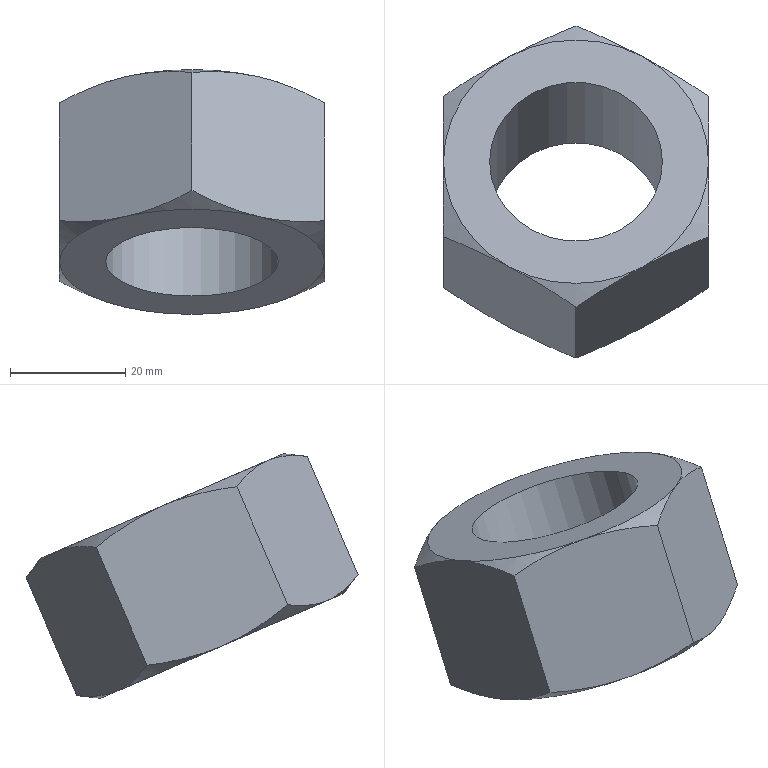Component | SolidWorks | hex nut gradec_iso-17 | 1 solid | 22 faces | box 46 x 57.6 x 42.45 mm | volume 29506 mm3 | cone 12 | plane 8 | cylinder 2 | commonest cylinder face diameters 30 x2
STEP:
#1=COLOUR_RGB('',0.7922,0.8196,0.9333);
#2=FILL_AREA_STYLE_COLOUR('',#1);
#3=FILL_AREA_STYLE('',(#2));
#4=SURFACE_STYLE_FILL_AREA(#3);
#5=SURFACE_SIDE_STYLE('',(#4));
#6=SURFACE_STYLE_USAGE(.BOTH.,#5);
#7=PRESENTATION_STYLE_ASSIGNMENT((#6));
#8=CARTESIAN_POINT('',(0.7087,-5.095,-11.818));
#9=VERTEX_POINT('',#8);
#10=CARTESIAN_POINT('',(1.89,-5.095,-11.818));
#11=VERTEX_POINT('',#10);
#12=CARTESIAN_POINT('',(1.299,-5.095,-11.818));
#13=DIRECTION('',(-0.,-0.3959,-0.9183));
#14=DIRECTION('',(1.,0.,0.));
#15=AXIS2_PLACEMENT_3D('',#12,#13,#14);
#16=CIRCLE('',#15,0.5906);
#17=EDGE_CURVE('',#9,#11,#16,.T.);
#18=ORIENTED_EDGE('',*,*,#17,.F.);
#19=CARTESIAN_POINT('',(0.7087,-5.507,-12.773));
#20=VERTEX_POINT('',#19);
#21=CARTESIAN_POINT('',(0.7087,-5.095,-11.818));
#22=DIRECTION('',(-0.,-0.3959,-0.9183));
#23=VECTOR('',#22,39.37);
#24=LINE('',#21,#23);
#25=EDGE_CURVE('',#9,#20,#24,.T.);
#26=ORIENTED_EDGE('',*,*,#25,.T.);
#27=CARTESIAN_POINT('',(1.89,-5.507,-12.773));
#28=VERTEX_POINT('',#27);
#29=CARTESIAN_POINT('',(1.299,-5.507,-12.773));
#30=DIRECTION('',(-0.,-0.3959,-0.9183));
#31=DIRECTION('',(1.,0.,0.));
#32=AXIS2_PLACEMENT_3D('',#29,#30,#31);
#33=CIRCLE('',#32,0.5906);
#34=EDGE_CURVE('',#20,#28,#33,.T.);
#35=ORIENTED_EDGE('',*,*,#34,.T.);
#36=CARTESIAN_POINT('',(1.89,-5.095,-11.818));
#37=DIRECTION('',(-0.,-0.3959,-0.9183));
#38=VECTOR('',#37,39.37);
#39=LINE('',#36,#38);
#40=EDGE_CURVE('',#11,#28,#39,.T.);
#41=ORIENTED_EDGE('',*,*,#40,.F.);
#42=EDGE_LOOP('',(#18,#26,#35,#41));
#43=FACE_OUTER_BOUND('',#42,.T.);
#44=CARTESIAN_POINT('',(1.299,-5.095,-11.818));
#45=DIRECTION('',(-0.,-0.3959,-0.9183));
#46=DIRECTION('',(1.,0.,0.));
#47=AXIS2_PLACEMENT_3D('',#44,#45,#46);
#48=CYLINDRICAL_SURFACE('',#47,0.5906);
#49=ADVANCED_FACE('',(#43),#48,.F.);
#50=CARTESIAN_POINT('',(0.3937,-5.607,-11.686));
#51=VERTEX_POINT('',#50);
#52=CARTESIAN_POINT('',(0.3937,-5.955,-12.492));
#53=VERTEX_POINT('',#52);
#54=CARTESIAN_POINT('',(0.3937,-5.575,-11.612));
#55=DIRECTION('',(-0.,-0.3959,-0.9183));
#56=VECTOR('',#55,39.37);
#57=LINE('',#54,#56);
#58=EDGE_CURVE('',#51,#53,#57,.T.);
#59=ORIENTED_EDGE('',*,*,#58,.T.);
#60=CARTESIAN_POINT('',(0.8465,-6.227,-12.462));
#61=VERTEX_POINT('',#60);
#62=CARTESIAN_POINT('',(0.3937,-5.955,-12.492));
#63=CARTESIAN_POINT('',(0.4678,-6.004,-12.497));
#64=CARTESIAN_POINT('',(0.5424,-6.052,-12.499));
#65=CARTESIAN_POINT('',(0.6931,-6.143,-12.49));
#66=CARTESIAN_POINT('',(0.7693,-6.186,-12.48));
#67=CARTESIAN_POINT('',(0.8465,-6.227,-12.462));
#68=B_SPLINE_CURVE_WITH_KNOTS('',3,(#62,#63,#64,#65,#66,#67),.UNSPECIFIED.,.F.,.F.,(4,2,4),(0.00000024,0.006718,0.01344),.UNSPECIFIED.);
#69=EDGE_CURVE('',#53,#61,#68,.T.);
#70=ORIENTED_EDGE('',*,*,#69,.T.);
#71=CARTESIAN_POINT('',(1.299,-6.435,-12.285));
#72=VERTEX_POINT('',#71);
#73=CARTESIAN_POINT('',(0.8465,-6.227,-12.462));
#74=CARTESIAN_POINT('',(0.8657,-6.237,-12.458));
#75=CARTESIAN_POINT('',(0.885,-6.247,-12.453));
#76=CARTESIAN_POINT('',(0.9234,-6.267,-12.443));
#77=CARTESIAN_POINT('',(0.9426,-6.276,-12.437));
#78=CARTESIAN_POINT('',(0.9998,-6.305,-12.419));
#79=CARTESIAN_POINT('',(1.038,-6.322,-12.405));
#80=CARTESIAN_POINT('',(1.151,-6.374,-12.36));
#81=CARTESIAN_POINT('',(1.225,-6.406,-12.324));
#82=CARTESIAN_POINT('',(1.299,-6.435,-12.285));
#83=B_SPLINE_CURVE_WITH_KNOTS('',3,(#73,#74,#75,#76,#77,#78,#79,#80,#81,#82),.UNSPECIFIED.,.F.,.F.,(4,2,2,2,4),(0.01344,0.01511,0.01678,0.02013,0.02682),.UNSPECIFIED.);
#84=EDGE_CURVE('',#61,#72,#83,.T.);
#85=ORIENTED_EDGE('',*,*,#84,.T.);
#86=CARTESIAN_POINT('',(1.299,-6.087,-11.479));
#87=VERTEX_POINT('',#86);
#88=CARTESIAN_POINT('',(1.299,-6.055,-11.405));
#89=DIRECTION('',(-0.,-0.3959,-0.9183));
#90=VECTOR('',#89,39.37);
#91=LINE('',#88,#90);
#92=EDGE_CURVE('',#87,#72,#91,.T.);
#93=ORIENTED_EDGE('',*,*,#92,.F.);
#94=CARTESIAN_POINT('',(0.8465,-5.815,-11.508));
#95=VERTEX_POINT('',#94);
#96=CARTESIAN_POINT('',(0.8465,-5.815,-11.508));
#97=CARTESIAN_POINT('',(0.8657,-5.826,-11.504));
#98=CARTESIAN_POINT('',(0.885,-5.836,-11.5));
#99=CARTESIAN_POINT('',(0.9234,-5.857,-11.493));
#100=CARTESIAN_POINT('',(0.9426,-5.868,-11.49));
#101=CARTESIAN_POINT('',(0.9998,-5.9,-11.482));
#102=CARTESIAN_POINT('',(1.038,-5.923,-11.478));
#103=CARTESIAN_POINT('',(1.151,-5.991,-11.471));
#104=CARTESIAN_POINT('',(1.225,-6.039,-11.473));
#105=CARTESIAN_POINT('',(1.299,-6.087,-11.479));
#106=B_SPLINE_CURVE_WITH_KNOTS('',3,(#96,#97,#98,#99,#100,#101,#102,#103,#104,#105),.UNSPECIFIED.,.F.,.F.,(4,2,2,2,4),(0.01344,0.01511,0.01678,0.02013,0.02682),.UNSPECIFIED.);
#107=EDGE_CURVE('',#95,#87,#106,.T.);
#108=ORIENTED_EDGE('',*,*,#107,.F.);
#109=CARTESIAN_POINT('',(0.3937,-5.607,-11.686));
#110=CARTESIAN_POINT('',(0.4678,-5.637,-11.646));
#111=CARTESIAN_POINT('',(0.5424,-5.668,-11.61));
#112=CARTESIAN_POINT('',(0.6931,-5.737,-11.55));
#113=CARTESIAN_POINT('',(0.7693,-5.775,-11.526));
#114=CARTESIAN_POINT('',(0.8465,-5.815,-11.508));
#115=B_SPLINE_CURVE_WITH_KNOTS('',3,(#109,#110,#111,#112,#113,#114),.UNSPECIFIED.,.F.,.F.,(4,2,4),(0.00000024,0.006718,0.01344),.UNSPECIFIED.);
#116=EDGE_CURVE('',#51,#95,#115,.T.);
#117=ORIENTED_EDGE('',*,*,#116,.F.);
#118=EDGE_LOOP('',(#59,#70,#85,#93,#108,#117));
#119=FACE_OUTER_BOUND('',#118,.T.);
#120=CARTESIAN_POINT('',(1.299,-6.055,-11.405));
#121=DIRECTION('',(-0.5,-0.7953,0.3429));
#122=DIRECTION('',(-0.866,0.4591,-0.198));
#123=AXIS2_PLACEMENT_3D('',#120,#121,#122);
#124=PLANE('',#123);
#125=ADVANCED_FACE('',(#119),#124,.T.);
#126=ORIENTED_EDGE('',*,*,#92,.T.);
#127=CARTESIAN_POINT('',(1.752,-6.227,-12.462));
#128=VERTEX_POINT('',#127);
#129=CARTESIAN_POINT('',(1.299,-6.435,-12.285));
#130=CARTESIAN_POINT('',(1.373,-6.405,-12.324));
#131=CARTESIAN_POINT('',(1.448,-6.374,-12.36));
#132=CARTESIAN_POINT('',(1.599,-6.305,-12.42));
#133=CARTESIAN_POINT('',(1.675,-6.268,-12.445));
#134=CARTESIAN_POINT('',(1.752,-6.227,-12.462));
#135=B_SPLINE_CURVE_WITH_KNOTS('',3,(#129,#130,#131,#132,#133,#134),.UNSPECIFIED.,.F.,.F.,(4,2,4),(0.00000024,0.006718,0.01344),.UNSPECIFIED.);
#136=EDGE_CURVE('',#72,#128,#135,.T.);
#137=ORIENTED_EDGE('',*,*,#136,.T.);
#138=CARTESIAN_POINT('',(2.205,-5.955,-12.492));
#139=VERTEX_POINT('',#138);
#140=CARTESIAN_POINT('',(1.752,-6.227,-12.462));
#141=CARTESIAN_POINT('',(1.771,-6.217,-12.467));
#142=CARTESIAN_POINT('',(1.79,-6.206,-12.471));
#143=CARTESIAN_POINT('',(1.829,-6.185,-12.478));
#144=CARTESIAN_POINT('',(1.848,-6.174,-12.481));
#145=CARTESIAN_POINT('',(1.905,-6.142,-12.489));
#146=CARTESIAN_POINT('',(1.943,-6.12,-12.493));
#147=CARTESIAN_POINT('',(2.056,-6.051,-12.499));
#148=CARTESIAN_POINT('',(2.131,-6.004,-12.497));
#149=CARTESIAN_POINT('',(2.205,-5.955,-12.492));
#150=B_SPLINE_CURVE_WITH_KNOTS('',3,(#140,#141,#142,#143,#144,#145,#146,#147,#148,#149),.UNSPECIFIED.,.F.,.F.,(4,2,2,2,4),(0.01344,0.01511,0.01678,0.02013,0.02682),.UNSPECIFIED.);
#151=EDGE_CURVE('',#128,#139,#150,.T.);
#152=ORIENTED_EDGE('',*,*,#151,.T.);
#153=CARTESIAN_POINT('',(2.205,-5.607,-11.686));
#154=VERTEX_POINT('',#153);
#155=CARTESIAN_POINT('',(2.205,-5.575,-11.612));
#156=DIRECTION('',(-0.,-0.3959,-0.9183));
#157=VECTOR('',#156,39.37);
#158=LINE('',#155,#157);
#159=EDGE_CURVE('',#154,#139,#158,.T.);
#160=ORIENTED_EDGE('',*,*,#159,.F.);
#161=CARTESIAN_POINT('',(1.752,-5.815,-11.508));
#162=VERTEX_POINT('',#161);
#163=CARTESIAN_POINT('',(1.752,-5.815,-11.508));
#164=CARTESIAN_POINT('',(1.771,-5.805,-11.512));
#165=CARTESIAN_POINT('',(1.79,-5.795,-11.517));
#166=CARTESIAN_POINT('',(1.829,-5.776,-11.528));
#167=CARTESIAN_POINT('',(1.848,-5.766,-11.533));
#168=CARTESIAN_POINT('',(1.905,-5.738,-11.552));
#169=CARTESIAN_POINT('',(1.943,-5.72,-11.565));
#170=CARTESIAN_POINT('',(2.056,-5.668,-11.611));
#171=CARTESIAN_POINT('',(2.131,-5.637,-11.646));
#172=CARTESIAN_POINT('',(2.205,-5.607,-11.686));
#173=B_SPLINE_CURVE_WITH_KNOTS('',3,(#163,#164,#165,#166,#167,#168,#169,#170,#171,#172),.UNSPECIFIED.,.F.,.F.,(4,2,2,2,4),(0.01344,0.01511,0.01678,0.02013,0.02682),.UNSPECIFIED.);
#174=EDGE_CURVE('',#162,#154,#173,.T.);
#175=ORIENTED_EDGE('',*,*,#174,.F.);
#176=CARTESIAN_POINT('',(1.299,-6.087,-11.479));
#177=CARTESIAN_POINT('',(1.373,-6.038,-11.473));
#178=CARTESIAN_POINT('',(1.448,-5.991,-11.471));
#179=CARTESIAN_POINT('',(1.599,-5.9,-11.48));
#180=CARTESIAN_POINT('',(1.675,-5.856,-11.49));
#181=CARTESIAN_POINT('',(1.752,-5.815,-11.508));
#182=B_SPLINE_CURVE_WITH_KNOTS('',3,(#176,#177,#178,#179,#180,#181),.UNSPECIFIED.,.F.,.F.,(4,2,4),(0.00000024,0.006718,0.01344),.UNSPECIFIED.);
#183=EDGE_CURVE('',#87,#162,#182,.T.);
#184=ORIENTED_EDGE('',*,*,#183,.F.);
#185=EDGE_LOOP('',(#126,#137,#152,#160,#175,#184));
#186=FACE_OUTER_BOUND('',#185,.T.);
#187=CARTESIAN_POINT('',(2.205,-5.575,-11.612));
#188=DIRECTION('',(0.5,-0.7953,0.3429));
#189=DIRECTION('',(-0.866,-0.4591,0.198));
#190=AXIS2_PLACEMENT_3D('',#187,#188,#189);
#191=PLANE('',#190);
#192=ADVANCED_FACE('',(#186),#191,.T.);
#193=CARTESIAN_POINT('',(2.205,-4.995,-12.906));
#194=VERTEX_POINT('',#193);
#195=CARTESIAN_POINT('',(2.205,-5.507,-12.773));
#196=VERTEX_POINT('',#195);
#197=CARTESIAN_POINT('',(2.205,-4.995,-12.906));
#198=CARTESIAN_POINT('',(2.205,-5.039,-12.9));
#199=CARTESIAN_POINT('',(2.205,-5.082,-12.893));
#200=CARTESIAN_POINT('',(2.205,-5.17,-12.877));
#201=CARTESIAN_POINT('',(2.205,-5.213,-12.868));
#202=CARTESIAN_POINT('',(2.205,-5.342,-12.836));
#203=CARTESIAN_POINT('',(2.205,-5.426,-12.808));
#204=CARTESIAN_POINT('',(2.205,-5.507,-12.773));
#205=B_SPLINE_CURVE_WITH_KNOTS('',3,(#197,#198,#199,#200,#201,#202,#203,#204),.UNSPECIFIED.,.F.,.F.,(4,2,2,4),(0.02369,0.02705,0.03041,0.03713),.UNSPECIFIED.);
#206=EDGE_CURVE('',#194,#196,#205,.T.);
#207=ORIENTED_EDGE('',*,*,#206,.F.);
#208=CARTESIAN_POINT('',(2.205,-4.647,-12.1));
#209=VERTEX_POINT('',#208);
#210=CARTESIAN_POINT('',(2.205,-4.615,-12.025));
#211=DIRECTION('',(-0.,-0.3959,-0.9183));
#212=VECTOR('',#211,39.37);
#213=LINE('',#210,#212);
#214=EDGE_CURVE('',#209,#194,#213,.T.);
#215=ORIENTED_EDGE('',*,*,#214,.F.);
#216=CARTESIAN_POINT('',(2.205,-5.095,-11.818));
#217=VERTEX_POINT('',#216);
#218=CARTESIAN_POINT('',(2.205,-4.647,-12.1));
#219=CARTESIAN_POINT('',(2.205,-4.681,-12.072));
#220=CARTESIAN_POINT('',(2.205,-4.716,-12.044));
#221=CARTESIAN_POINT('',(2.205,-4.788,-11.992));
#222=CARTESIAN_POINT('',(2.205,-4.825,-11.966));
#223=CARTESIAN_POINT('',(2.205,-4.937,-11.895));
#224=CARTESIAN_POINT('',(2.205,-5.014,-11.853));
#225=CARTESIAN_POINT('',(2.205,-5.095,-11.818));
#226=B_SPLINE_CURVE_WITH_KNOTS('',3,(#218,#219,#220,#221,#222,#223,#224,#225),.UNSPECIFIED.,.F.,.F.,(4,2,2,4),(0.02369,0.02705,0.03041,0.03713),.UNSPECIFIED.);
#227=EDGE_CURVE('',#209,#217,#226,.T.);
#228=ORIENTED_EDGE('',*,*,#227,.T.);
#229=CARTESIAN_POINT('',(2.205,-5.095,-11.818));
#230=CARTESIAN_POINT('',(2.205,-5.136,-11.801));
#231=CARTESIAN_POINT('',(2.205,-5.177,-11.785));
#232=CARTESIAN_POINT('',(2.205,-5.262,-11.757));
#233=CARTESIAN_POINT('',(2.205,-5.305,-11.744));
#234=CARTESIAN_POINT('',(2.205,-5.433,-11.712));
#235=CARTESIAN_POINT('',(2.205,-5.52,-11.697));
#236=CARTESIAN_POINT('',(2.205,-5.607,-11.686));
#237=B_SPLINE_CURVE_WITH_KNOTS('',3,(#229,#230,#231,#232,#233,#234,#235,#236),.UNSPECIFIED.,.F.,.F.,(4,2,2,4),(0.03713,0.04049,0.04385,0.05057),.UNSPECIFIED.);
#238=EDGE_CURVE('',#217,#154,#237,.T.);
#239=ORIENTED_EDGE('',*,*,#238,.T.);
#240=ORIENTED_EDGE('',*,*,#159,.T.);
#241=CARTESIAN_POINT('',(2.205,-5.507,-12.773));
#242=CARTESIAN_POINT('',(2.205,-5.547,-12.755));
#243=CARTESIAN_POINT('',(2.205,-5.587,-12.736));
#244=CARTESIAN_POINT('',(2.205,-5.666,-12.694));
#245=CARTESIAN_POINT('',(2.205,-5.704,-12.672));
#246=CARTESIAN_POINT('',(2.205,-5.816,-12.6));
#247=CARTESIAN_POINT('',(2.205,-5.887,-12.548));
#248=CARTESIAN_POINT('',(2.205,-5.955,-12.492));
#249=B_SPLINE_CURVE_WITH_KNOTS('',3,(#241,#242,#243,#244,#245,#246,#247,#248),.UNSPECIFIED.,.F.,.F.,(4,2,2,4),(0.03713,0.04049,0.04385,0.05057),.UNSPECIFIED.);
#250=EDGE_CURVE('',#196,#139,#249,.T.);
#251=ORIENTED_EDGE('',*,*,#250,.F.);
#252=EDGE_LOOP('',(#207,#215,#228,#239,#240,#251));
#253=FACE_OUTER_BOUND('',#252,.T.);
#254=CARTESIAN_POINT('',(2.205,-5.575,-11.612));
#255=DIRECTION('',(-1.,0.,-0.));
#256=DIRECTION('',(-0.,-0.3959,-0.9183));
#257=AXIS2_PLACEMENT_3D('',#254,#255,#256);
#258=PLANE('',#257);
#259=ADVANCED_FACE('',(#253),#258,.F.);
#260=ORIENTED_EDGE('',*,*,#214,.T.);
#261=CARTESIAN_POINT('',(1.752,-4.787,-13.083));
#262=VERTEX_POINT('',#261);
#263=CARTESIAN_POINT('',(2.205,-4.995,-12.906));
#264=CARTESIAN_POINT('',(2.131,-4.965,-12.945));
#265=CARTESIAN_POINT('',(2.056,-4.934,-12.981));
#266=CARTESIAN_POINT('',(1.905,-4.865,-13.041));
#267=CARTESIAN_POINT('',(1.829,-4.828,-13.066));
#268=CARTESIAN_POINT('',(1.752,-4.787,-13.083));
#269=B_SPLINE_CURVE_WITH_KNOTS('',3,(#263,#264,#265,#266,#267,#268),.UNSPECIFIED.,.F.,.F.,(4,2,4),(0.00000024,0.006718,0.01344),.UNSPECIFIED.);
#270=EDGE_CURVE('',#194,#262,#269,.T.);
#271=ORIENTED_EDGE('',*,*,#270,.T.);
#272=CARTESIAN_POINT('',(1.299,-4.515,-13.113));
#273=VERTEX_POINT('',#272);
#274=CARTESIAN_POINT('',(1.752,-4.787,-13.083));
#275=CARTESIAN_POINT('',(1.733,-4.776,-13.088));
#276=CARTESIAN_POINT('',(1.713,-4.766,-13.092));
#277=CARTESIAN_POINT('',(1.675,-4.745,-13.099));
#278=CARTESIAN_POINT('',(1.656,-4.734,-13.102));
#279=CARTESIAN_POINT('',(1.599,-4.702,-13.11));
#280=CARTESIAN_POINT('',(1.561,-4.679,-13.114));
#281=CARTESIAN_POINT('',(1.448,-4.611,-13.12));
#282=CARTESIAN_POINT('',(1.373,-4.564,-13.118));
#283=CARTESIAN_POINT('',(1.299,-4.515,-13.113));
#284=B_SPLINE_CURVE_WITH_KNOTS('',3,(#274,#275,#276,#277,#278,#279,#280,#281,#282,#283),.UNSPECIFIED.,.F.,.F.,(4,2,2,2,4),(0.01344,0.01511,0.01678,0.02013,0.02682),.UNSPECIFIED.);
#285=EDGE_CURVE('',#262,#273,#284,.T.);
#286=ORIENTED_EDGE('',*,*,#285,.T.);
#287=CARTESIAN_POINT('',(1.299,-4.167,-12.307));
#288=VERTEX_POINT('',#287);
#289=CARTESIAN_POINT('',(1.299,-4.135,-12.232));
#290=DIRECTION('',(-0.,-0.3959,-0.9183));
#291=VECTOR('',#290,39.37);
#292=LINE('',#289,#291);
#293=EDGE_CURVE('',#288,#273,#292,.T.);
#294=ORIENTED_EDGE('',*,*,#293,.F.);
#295=CARTESIAN_POINT('',(1.752,-4.375,-12.129));
#296=VERTEX_POINT('',#295);
#297=CARTESIAN_POINT('',(1.752,-4.375,-12.129));
#298=CARTESIAN_POINT('',(1.733,-4.365,-12.133));
#299=CARTESIAN_POINT('',(1.713,-4.355,-12.138));
#300=CARTESIAN_POINT('',(1.675,-4.335,-12.149));
#301=CARTESIAN_POINT('',(1.656,-4.326,-12.154));
#302=CARTESIAN_POINT('',(1.599,-4.298,-12.173));
#303=CARTESIAN_POINT('',(1.561,-4.28,-12.186));
#304=CARTESIAN_POINT('',(1.448,-4.228,-12.232));
#305=CARTESIAN_POINT('',(1.373,-4.197,-12.267));
#306=CARTESIAN_POINT('',(1.299,-4.167,-12.307));
#307=B_SPLINE_CURVE_WITH_KNOTS('',3,(#297,#298,#299,#300,#301,#302,#303,#304,#305,#306),.UNSPECIFIED.,.F.,.F.,(4,2,2,2,4),(0.01344,0.01511,0.01678,0.02013,0.02682),.UNSPECIFIED.);
#308=EDGE_CURVE('',#296,#288,#307,.T.);
#309=ORIENTED_EDGE('',*,*,#308,.F.);
#310=CARTESIAN_POINT('',(2.205,-4.647,-12.1));
#311=CARTESIAN_POINT('',(2.131,-4.598,-12.094));
#312=CARTESIAN_POINT('',(2.056,-4.551,-12.092));
#313=CARTESIAN_POINT('',(1.905,-4.46,-12.101));
#314=CARTESIAN_POINT('',(1.829,-4.416,-12.111));
#315=CARTESIAN_POINT('',(1.752,-4.375,-12.129));
#316=B_SPLINE_CURVE_WITH_KNOTS('',3,(#310,#311,#312,#313,#314,#315),.UNSPECIFIED.,.F.,.F.,(4,2,4),(0.00000024,0.006718,0.01344),.UNSPECIFIED.);
#317=EDGE_CURVE('',#209,#296,#316,.T.);
#318=ORIENTED_EDGE('',*,*,#317,.F.);
#319=EDGE_LOOP('',(#260,#271,#286,#294,#309,#318));
#320=FACE_OUTER_BOUND('',#319,.T.);
#321=CARTESIAN_POINT('',(1.299,-4.135,-12.232));
#322=DIRECTION('',(0.5,0.7953,-0.3429));
#323=DIRECTION('',(0.866,-0.4591,0.198));
#324=AXIS2_PLACEMENT_3D('',#321,#322,#323);
#325=PLANE('',#324);
#326=ADVANCED_FACE('',(#320),#325,.T.);
#327=ORIENTED_EDGE('',*,*,#293,.T.);
#328=CARTESIAN_POINT('',(0.8465,-4.787,-13.083));
#329=VERTEX_POINT('',#328);
#330=CARTESIAN_POINT('',(1.299,-4.515,-13.113));
#331=CARTESIAN_POINT('',(1.225,-4.564,-13.118));
#332=CARTESIAN_POINT('',(1.151,-4.611,-13.12));
#333=CARTESIAN_POINT('',(0.9998,-4.702,-13.111));
#334=CARTESIAN_POINT('',(0.9236,-4.746,-13.101));
#335=CARTESIAN_POINT('',(0.8465,-4.787,-13.083));
#336=B_SPLINE_CURVE_WITH_KNOTS('',3,(#330,#331,#332,#333,#334,#335),.UNSPECIFIED.,.F.,.F.,(4,2,4),(0.00000024,0.006718,0.01344),.UNSPECIFIED.);
#337=EDGE_CURVE('',#273,#329,#336,.T.);
#338=ORIENTED_EDGE('',*,*,#337,.T.);
#339=CARTESIAN_POINT('',(0.3937,-4.995,-12.906));
#340=VERTEX_POINT('',#339);
#341=CARTESIAN_POINT('',(0.8465,-4.787,-13.083));
#342=CARTESIAN_POINT('',(0.8272,-4.797,-13.079));
#343=CARTESIAN_POINT('',(0.8079,-4.807,-13.074));
#344=CARTESIAN_POINT('',(0.7695,-4.827,-13.064));
#345=CARTESIAN_POINT('',(0.7503,-4.836,-13.058));
#346=CARTESIAN_POINT('',(0.6931,-4.864,-13.04));
#347=CARTESIAN_POINT('',(0.6552,-4.882,-13.026));
#348=CARTESIAN_POINT('',(0.5421,-4.934,-12.981));
#349=CARTESIAN_POINT('',(0.4676,-4.965,-12.945));
#350=CARTESIAN_POINT('',(0.3937,-4.995,-12.906));
#351=B_SPLINE_CURVE_WITH_KNOTS('',3,(#341,#342,#343,#344,#345,#346,#347,#348,#349,#350),.UNSPECIFIED.,.F.,.F.,(4,2,2,2,4),(0.01344,0.01511,0.01678,0.02013,0.02682),.UNSPECIFIED.);
#352=EDGE_CURVE('',#329,#340,#351,.T.);
#353=ORIENTED_EDGE('',*,*,#352,.T.);
#354=CARTESIAN_POINT('',(0.3937,-4.647,-12.1));
#355=VERTEX_POINT('',#354);
#356=CARTESIAN_POINT('',(0.3937,-4.615,-12.025));
#357=DIRECTION('',(-0.,-0.3959,-0.9183));
#358=VECTOR('',#357,39.37);
#359=LINE('',#356,#358);
#360=EDGE_CURVE('',#355,#340,#359,.T.);
#361=ORIENTED_EDGE('',*,*,#360,.F.);
#362=CARTESIAN_POINT('',(0.8465,-4.375,-12.129));
#363=VERTEX_POINT('',#362);
#364=CARTESIAN_POINT('',(0.8465,-4.375,-12.129));
#365=CARTESIAN_POINT('',(0.8272,-4.385,-12.125));
#366=CARTESIAN_POINT('',(0.8079,-4.396,-12.121));
#367=CARTESIAN_POINT('',(0.7695,-4.417,-12.114));
#368=CARTESIAN_POINT('',(0.7503,-4.428,-12.11));
#369=CARTESIAN_POINT('',(0.6931,-4.46,-12.102));
#370=CARTESIAN_POINT('',(0.6552,-4.482,-12.099));
#371=CARTESIAN_POINT('',(0.5421,-4.551,-12.092));
#372=CARTESIAN_POINT('',(0.4676,-4.598,-12.094));
#373=CARTESIAN_POINT('',(0.3937,-4.647,-12.1));
#374=B_SPLINE_CURVE_WITH_KNOTS('',3,(#364,#365,#366,#367,#368,#369,#370,#371,#372,#373),.UNSPECIFIED.,.F.,.F.,(4,2,2,2,4),(0.01344,0.01511,0.01678,0.02013,0.02682),.UNSPECIFIED.);
#375=EDGE_CURVE('',#363,#355,#374,.T.);
#376=ORIENTED_EDGE('',*,*,#375,.F.);
#377=CARTESIAN_POINT('',(1.299,-4.167,-12.307));
#378=CARTESIAN_POINT('',(1.225,-4.197,-12.267));
#379=CARTESIAN_POINT('',(1.151,-4.228,-12.231));
#380=CARTESIAN_POINT('',(0.9998,-4.297,-12.171));
#381=CARTESIAN_POINT('',(0.9236,-4.334,-12.147));
#382=CARTESIAN_POINT('',(0.8465,-4.375,-12.129));
#383=B_SPLINE_CURVE_WITH_KNOTS('',3,(#377,#378,#379,#380,#381,#382),.UNSPECIFIED.,.F.,.F.,(4,2,4),(0.00000024,0.006718,0.01344),.UNSPECIFIED.);
#384=EDGE_CURVE('',#288,#363,#383,.T.);
#385=ORIENTED_EDGE('',*,*,#384,.F.);
#386=EDGE_LOOP('',(#327,#338,#353,#361,#376,#385));
#387=FACE_OUTER_BOUND('',#386,.T.);
#388=CARTESIAN_POINT('',(0.3937,-4.615,-12.025));
#389=DIRECTION('',(-0.5,0.7953,-0.3429));
#390=DIRECTION('',(0.866,0.4591,-0.198));
#391=AXIS2_PLACEMENT_3D('',#388,#389,#390);
#392=PLANE('',#391);
#393=ADVANCED_FACE('',(#387),#392,.T.);
#394=ORIENTED_EDGE('',*,*,#360,.T.);
#395=CARTESIAN_POINT('',(0.3937,-5.507,-12.773));
#396=VERTEX_POINT('',#395);
#397=CARTESIAN_POINT('',(0.3937,-4.995,-12.906));
#398=CARTESIAN_POINT('',(0.3937,-5.039,-12.9));
#399=CARTESIAN_POINT('',(0.3937,-5.082,-12.893));
#400=CARTESIAN_POINT('',(0.3937,-5.17,-12.877));
#401=CARTESIAN_POINT('',(0.3937,-5.213,-12.868));
#402=CARTESIAN_POINT('',(0.3937,-5.342,-12.836));
#403=CARTESIAN_POINT('',(0.3937,-5.426,-12.808));
#404=CARTESIAN_POINT('',(0.3937,-5.507,-12.773));
#405=B_SPLINE_CURVE_WITH_KNOTS('',3,(#397,#398,#399,#400,#401,#402,#403,#404),.UNSPECIFIED.,.F.,.F.,(4,2,2,4),(0.02369,0.02705,0.03041,0.03713),.UNSPECIFIED.);
#406=EDGE_CURVE('',#340,#396,#405,.T.);
#407=ORIENTED_EDGE('',*,*,#406,.T.);
#408=CARTESIAN_POINT('',(0.3937,-5.507,-12.773));
#409=CARTESIAN_POINT('',(0.3937,-5.547,-12.755));
#410=CARTESIAN_POINT('',(0.3937,-5.587,-12.736));
#411=CARTESIAN_POINT('',(0.3937,-5.666,-12.694));
#412=CARTESIAN_POINT('',(0.3937,-5.704,-12.672));
#413=CARTESIAN_POINT('',(0.3937,-5.816,-12.6));
#414=CARTESIAN_POINT('',(0.3937,-5.887,-12.548));
#415=CARTESIAN_POINT('',(0.3937,-5.955,-12.492));
#416=B_SPLINE_CURVE_WITH_KNOTS('',3,(#408,#409,#410,#411,#412,#413,#414,#415),.UNSPECIFIED.,.F.,.F.,(4,2,2,4),(0.03713,0.04049,0.04385,0.05057),.UNSPECIFIED.);
#417=EDGE_CURVE('',#396,#53,#416,.T.);
#418=ORIENTED_EDGE('',*,*,#417,.T.);
#419=ORIENTED_EDGE('',*,*,#58,.F.);
#420=CARTESIAN_POINT('',(0.3937,-5.095,-11.818));
#421=VERTEX_POINT('',#420);
#422=CARTESIAN_POINT('',(0.3937,-5.095,-11.818));
#423=CARTESIAN_POINT('',(0.3937,-5.136,-11.801));
#424=CARTESIAN_POINT('',(0.3937,-5.177,-11.785));
#425=CARTESIAN_POINT('',(0.3937,-5.262,-11.757));
#426=CARTESIAN_POINT('',(0.3937,-5.305,-11.744));
#427=CARTESIAN_POINT('',(0.3937,-5.433,-11.712));
#428=CARTESIAN_POINT('',(0.3937,-5.52,-11.697));
#429=CARTESIAN_POINT('',(0.3937,-5.607,-11.686));
#430=B_SPLINE_CURVE_WITH_KNOTS('',3,(#422,#423,#424,#425,#426,#427,#428,#429),.UNSPECIFIED.,.F.,.F.,(4,2,2,4),(0.03713,0.04049,0.04385,0.05057),.UNSPECIFIED.);
#431=EDGE_CURVE('',#421,#51,#430,.T.);
#432=ORIENTED_EDGE('',*,*,#431,.F.);
#433=CARTESIAN_POINT('',(0.3937,-4.647,-12.1));
#434=CARTESIAN_POINT('',(0.3937,-4.681,-12.072));
#435=CARTESIAN_POINT('',(0.3937,-4.716,-12.044));
#436=CARTESIAN_POINT('',(0.3937,-4.788,-11.992));
#437=CARTESIAN_POINT('',(0.3937,-4.825,-11.966));
#438=CARTESIAN_POINT('',(0.3937,-4.937,-11.895));
#439=CARTESIAN_POINT('',(0.3937,-5.014,-11.853));
#440=CARTESIAN_POINT('',(0.3937,-5.095,-11.818));
#441=B_SPLINE_CURVE_WITH_KNOTS('',3,(#433,#434,#435,#436,#437,#438,#439,#440),.UNSPECIFIED.,.F.,.F.,(4,2,2,4),(0.02369,0.02705,0.03041,0.03713),.UNSPECIFIED.);
#442=EDGE_CURVE('',#355,#421,#441,.T.);
#443=ORIENTED_EDGE('',*,*,#442,.F.);
#444=EDGE_LOOP('',(#394,#407,#418,#419,#432,#443));
#445=FACE_OUTER_BOUND('',#444,.T.);
#446=CARTESIAN_POINT('',(0.3937,-5.575,-11.612));
#447=DIRECTION('',(-1.,0.,-0.));
#448=DIRECTION('',(-0.,-0.3959,-0.9183));
#449=AXIS2_PLACEMENT_3D('',#446,#447,#448);
#450=PLANE('',#449);
#451=ADVANCED_FACE('',(#445),#450,.T.);
#452=CARTESIAN_POINT('',(1.299,-5.507,-12.773));
#453=DIRECTION('',(-0.,-0.3959,-0.9183));
#454=DIRECTION('',(1.,0.,0.));
#455=AXIS2_PLACEMENT_3D('',#452,#453,#454);
#456=CIRCLE('',#455,0.5906);
#457=EDGE_CURVE('',#28,#20,#456,.T.);
#458=ORIENTED_EDGE('',*,*,#457,.F.);
#459=ORIENTED_EDGE('',*,*,#34,.F.);
#460=EDGE_LOOP('',(#458,#459));
#461=FACE_BOUND('',#460,.T.);
#462=CARTESIAN_POINT('',(1.299,-5.507,-12.773));
#463=DIRECTION('',(-0.,-0.3959,-0.9183));
#464=DIRECTION('',(1.,-0.,0.));
#465=AXIS2_PLACEMENT_3D('',#462,#463,#464);
#466=CIRCLE('',#465,0.9055);
#467=EDGE_CURVE('',#262,#196,#466,.T.);
#468=ORIENTED_EDGE('',*,*,#467,.T.);
#469=CARTESIAN_POINT('',(1.299,-5.507,-12.773));
#470=DIRECTION('',(-0.,-0.3959,-0.9183));
#471=DIRECTION('',(1.,-0.,0.));
#472=AXIS2_PLACEMENT_3D('',#469,#470,#471);
#473=CIRCLE('',#472,0.9055);
#474=EDGE_CURVE('',#196,#128,#473,.T.);
#475=ORIENTED_EDGE('',*,*,#474,.T.);
#476=CARTESIAN_POINT('',(1.299,-5.507,-12.773));
#477=DIRECTION('',(-0.,-0.3959,-0.9183));
#478=DIRECTION('',(1.,-0.,0.));
#479=AXIS2_PLACEMENT_3D('',#476,#477,#478);
#480=CIRCLE('',#479,0.9055);
#481=EDGE_CURVE('',#128,#61,#480,.T.);
#482=ORIENTED_EDGE('',*,*,#481,.T.);
#483=CARTESIAN_POINT('',(1.299,-5.507,-12.773));
#484=DIRECTION('',(-0.,-0.3959,-0.9183));
#485=DIRECTION('',(1.,-0.,0.));
#486=AXIS2_PLACEMENT_3D('',#483,#484,#485);
#487=CIRCLE('',#486,0.9055);
#488=EDGE_CURVE('',#61,#396,#487,.T.);
#489=ORIENTED_EDGE('',*,*,#488,.T.);
#490=CARTESIAN_POINT('',(1.299,-5.507,-12.773));
#491=DIRECTION('',(-0.,-0.3959,-0.9183));
#492=DIRECTION('',(1.,-0.,0.));
#493=AXIS2_PLACEMENT_3D('',#490,#491,#492);
#494=CIRCLE('',#493,0.9055);
#495=EDGE_CURVE('',#396,#329,#494,.T.);
#496=ORIENTED_EDGE('',*,*,#495,.T.);
#497=CARTESIAN_POINT('',(1.299,-5.507,-12.773));
#498=DIRECTION('',(-0.,-0.3959,-0.9183));
#499=DIRECTION('',(1.,-0.,0.));
#500=AXIS2_PLACEMENT_3D('',#497,#498,#499);
#501=CIRCLE('',#500,0.9055);
#502=EDGE_CURVE('',#329,#262,#501,.T.);
#503=ORIENTED_EDGE('',*,*,#502,.T.);
#504=EDGE_LOOP('',(#468,#475,#482,#489,#496,#503));
#505=FACE_OUTER_BOUND('',#504,.T.);
#506=CARTESIAN_POINT('',(-0.5118,-5.507,-12.773));
#507=DIRECTION('',(-0.,-0.3959,-0.9183));
#508=DIRECTION('',(1.,-0.,0.));
#509=AXIS2_PLACEMENT_3D('',#506,#507,#508);
#510=PLANE('',#509);
#511=ADVANCED_FACE('',(#461,#505),#510,.T.);
#512=CARTESIAN_POINT('',(1.299,-5.095,-11.818));
#513=DIRECTION('',(-0.,-0.3959,-0.9183));
#514=DIRECTION('',(1.,0.,0.));
#515=AXIS2_PLACEMENT_3D('',#512,#513,#514);
#516=CIRCLE('',#515,0.5906);
#517=EDGE_CURVE('',#11,#9,#516,.T.);
#518=ORIENTED_EDGE('',*,*,#517,.T.);
#519=ORIENTED_EDGE('',*,*,#17,.T.);
#520=EDGE_LOOP('',(#518,#519));
#521=FACE_BOUND('',#520,.T.);
#522=CARTESIAN_POINT('',(1.299,-5.095,-11.818));
#523=DIRECTION('',(-0.,-0.3959,-0.9183));
#524=DIRECTION('',(1.,-0.,0.));
#525=AXIS2_PLACEMENT_3D('',#522,#523,#524);
#526=CIRCLE('',#525,0.9055);
#527=EDGE_CURVE('',#217,#162,#526,.T.);
#528=ORIENTED_EDGE('',*,*,#527,.F.);
#529=CARTESIAN_POINT('',(1.299,-5.095,-11.818));
#530=DIRECTION('',(0.,0.3959,0.9183));
#531=DIRECTION('',(1.,-0.,0.));
#532=AXIS2_PLACEMENT_3D('',#529,#530,#531);
#533=CIRCLE('',#532,0.9055);
#534=EDGE_CURVE('',#217,#296,#533,.T.);
#535=ORIENTED_EDGE('',*,*,#534,.T.);
#536=CARTESIAN_POINT('',(1.299,-5.095,-11.818));
#537=DIRECTION('',(0.,0.3959,0.9183));
#538=DIRECTION('',(1.,-0.,0.));
#539=AXIS2_PLACEMENT_3D('',#536,#537,#538);
#540=CIRCLE('',#539,0.9055);
#541=EDGE_CURVE('',#296,#363,#540,.T.);
#542=ORIENTED_EDGE('',*,*,#541,.T.);
#543=CARTESIAN_POINT('',(1.299,-5.095,-11.818));
#544=DIRECTION('',(0.,0.3959,0.9183));
#545=DIRECTION('',(1.,0.,0.));
#546=AXIS2_PLACEMENT_3D('',#543,#544,#545);
#547=CIRCLE('',#546,0.9055);
#548=EDGE_CURVE('',#363,#421,#547,.T.);
#549=ORIENTED_EDGE('',*,*,#548,.T.);
#550=CARTESIAN_POINT('',(1.299,-5.095,-11.818));
#551=DIRECTION('',(0.,0.3959,0.9183));
#552=DIRECTION('',(1.,-0.,0.));
#553=AXIS2_PLACEMENT_3D('',#550,#551,#552);
#554=CIRCLE('',#553,0.9055);
#555=EDGE_CURVE('',#421,#95,#554,.T.);
#556=ORIENTED_EDGE('',*,*,#555,.T.);
#557=CARTESIAN_POINT('',(1.299,-5.095,-11.818));
#558=DIRECTION('',(0.,0.3959,0.9183));
#559=DIRECTION('',(1.,0.,0.));
#560=AXIS2_PLACEMENT_3D('',#557,#558,#559);
#561=CIRCLE('',#560,0.9055);
#562=EDGE_CURVE('',#95,#162,#561,.T.);
#563=ORIENTED_EDGE('',*,*,#562,.T.);
#564=EDGE_LOOP('',(#528,#535,#542,#549,#556,#563));
#565=FACE_OUTER_BOUND('',#564,.T.);
#566=CARTESIAN_POINT('',(-0.5118,-5.095,-11.818));
#567=DIRECTION('',(-0.,-0.3959,-0.9183));
#568=DIRECTION('',(1.,-0.,0.));
#569=AXIS2_PLACEMENT_3D('',#566,#567,#568);
#570=PLANE('',#569);
#571=ADVANCED_FACE('',(#521,#565),#570,.F.);
#572=ORIENTED_EDGE('',*,*,#25,.F.);
#573=ORIENTED_EDGE('',*,*,#517,.F.);
#574=ORIENTED_EDGE('',*,*,#40,.T.);
#575=ORIENTED_EDGE('',*,*,#457,.T.);
#576=EDGE_LOOP('',(#572,#573,#574,#575));
#577=FACE_OUTER_BOUND('',#576,.T.);
#578=CARTESIAN_POINT('',(1.299,-5.095,-11.818));
#579=DIRECTION('',(-0.,-0.3959,-0.9183));
#580=DIRECTION('',(1.,0.,0.));
#581=AXIS2_PLACEMENT_3D('',#578,#579,#580);
#582=CYLINDRICAL_SURFACE('',#581,0.5906);
#583=ADVANCED_FACE('',(#577),#582,.F.);
#584=ORIENTED_EDGE('',*,*,#174,.T.);
#585=ORIENTED_EDGE('',*,*,#238,.F.);
#586=ORIENTED_EDGE('',*,*,#527,.T.);
#587=EDGE_LOOP('',(#584,#585,#586));
#588=FACE_OUTER_BOUND('',#587,.T.);
#589=CARTESIAN_POINT('',(1.299,-5.095,-11.818));
#590=DIRECTION('',(-0.,-0.3959,-0.9183));
#591=DIRECTION('',(1.,-0.,0.));
#592=AXIS2_PLACEMENT_3D('',#589,#590,#591);
#593=CONICAL_SURFACE('',#592,0.9055,1.047);
#594=ADVANCED_FACE('',(#588),#593,.T.);
#595=ORIENTED_EDGE('',*,*,#107,.T.);
#596=ORIENTED_EDGE('',*,*,#183,.T.);
#597=ORIENTED_EDGE('',*,*,#562,.F.);
#598=EDGE_LOOP('',(#595,#596,#597));
#599=FACE_OUTER_BOUND('',#598,.T.);
#600=CARTESIAN_POINT('',(1.299,-5.095,-11.818));
#601=DIRECTION('',(-0.,-0.3959,-0.9183));
#602=DIRECTION('',(1.,-0.,0.));
#603=AXIS2_PLACEMENT_3D('',#600,#601,#602);
#604=CONICAL_SURFACE('',#603,0.9055,1.047);
#605=ADVANCED_FACE('',(#599),#604,.T.);
#606=ORIENTED_EDGE('',*,*,#116,.T.);
#607=ORIENTED_EDGE('',*,*,#555,.F.);
#608=ORIENTED_EDGE('',*,*,#431,.T.);
#609=EDGE_LOOP('',(#606,#607,#608));
#610=FACE_OUTER_BOUND('',#609,.T.);
#611=CARTESIAN_POINT('',(1.299,-5.095,-11.818));
#612=DIRECTION('',(-0.,-0.3959,-0.9183));
#613=DIRECTION('',(1.,-0.,0.));
#614=AXIS2_PLACEMENT_3D('',#611,#612,#613);
#615=CONICAL_SURFACE('',#614,0.9055,1.047);
#616=ADVANCED_FACE('',(#610),#615,.T.);
#617=ORIENTED_EDGE('',*,*,#375,.T.);
#618=ORIENTED_EDGE('',*,*,#442,.T.);
#619=ORIENTED_EDGE('',*,*,#548,.F.);
#620=EDGE_LOOP('',(#617,#618,#619));
#621=FACE_OUTER_BOUND('',#620,.T.);
#622=CARTESIAN_POINT('',(1.299,-5.095,-11.818));
#623=DIRECTION('',(-0.,-0.3959,-0.9183));
#624=DIRECTION('',(1.,-0.,0.));
#625=AXIS2_PLACEMENT_3D('',#622,#623,#624);
#626=CONICAL_SURFACE('',#625,0.9055,1.047);
#627=ADVANCED_FACE('',(#621),#626,.T.);
#628=ORIENTED_EDGE('',*,*,#308,.T.);
#629=ORIENTED_EDGE('',*,*,#384,.T.);
#630=ORIENTED_EDGE('',*,*,#541,.F.);
#631=EDGE_LOOP('',(#628,#629,#630));
#632=FACE_OUTER_BOUND('',#631,.T.);
#633=CARTESIAN_POINT('',(1.299,-5.095,-11.818));
#634=DIRECTION('',(-0.,-0.3959,-0.9183));
#635=DIRECTION('',(1.,-0.,0.));
#636=AXIS2_PLACEMENT_3D('',#633,#634,#635);
#637=CONICAL_SURFACE('',#636,0.9055,1.047);
#638=ADVANCED_FACE('',(#632),#637,.T.);
#639=ORIENTED_EDGE('',*,*,#317,.T.);
#640=ORIENTED_EDGE('',*,*,#534,.F.);
#641=ORIENTED_EDGE('',*,*,#227,.F.);
#642=EDGE_LOOP('',(#639,#640,#641));
#643=FACE_OUTER_BOUND('',#642,.T.);
#644=CARTESIAN_POINT('',(1.299,-5.095,-11.818));
#645=DIRECTION('',(-0.,-0.3959,-0.9183));
#646=DIRECTION('',(1.,-0.,0.));
#647=AXIS2_PLACEMENT_3D('',#644,#645,#646);
#648=CONICAL_SURFACE('',#647,0.9055,1.047);
#649=ADVANCED_FACE('',(#643),#648,.T.);
#650=ORIENTED_EDGE('',*,*,#206,.T.);
#651=ORIENTED_EDGE('',*,*,#467,.F.);
#652=ORIENTED_EDGE('',*,*,#270,.F.);
#653=EDGE_LOOP('',(#650,#651,#652));
#654=FACE_OUTER_BOUND('',#653,.T.);
#655=CARTESIAN_POINT('',(1.299,-5.507,-12.773));
#656=DIRECTION('',(0.,0.3959,0.9183));
#657=DIRECTION('',(-1.,0.,0.));
#658=AXIS2_PLACEMENT_3D('',#655,#656,#657);
#659=CONICAL_SURFACE('',#658,0.9055,1.047);
#660=ADVANCED_FACE('',(#654),#659,.T.);
#661=ORIENTED_EDGE('',*,*,#502,.F.);
#662=ORIENTED_EDGE('',*,*,#337,.F.);
#663=ORIENTED_EDGE('',*,*,#285,.F.);
#664=EDGE_LOOP('',(#661,#662,#663));
#665=FACE_OUTER_BOUND('',#664,.T.);
#666=CARTESIAN_POINT('',(1.299,-5.507,-12.773));
#667=DIRECTION('',(0.,0.3959,0.9183));
#668=DIRECTION('',(-1.,0.,0.));
#669=AXIS2_PLACEMENT_3D('',#666,#667,#668);
#670=CONICAL_SURFACE('',#669,0.9055,1.047);
#671=ADVANCED_FACE('',(#665),#670,.T.);
#672=ORIENTED_EDGE('',*,*,#495,.F.);
#673=ORIENTED_EDGE('',*,*,#406,.F.);
#674=ORIENTED_EDGE('',*,*,#352,.F.);
#675=EDGE_LOOP('',(#672,#673,#674));
#676=FACE_OUTER_BOUND('',#675,.T.);
#677=CARTESIAN_POINT('',(1.299,-5.507,-12.773));
#678=DIRECTION('',(0.,0.3959,0.9183));
#679=DIRECTION('',(-1.,0.,0.));
#680=AXIS2_PLACEMENT_3D('',#677,#678,#679);
#681=CONICAL_SURFACE('',#680,0.9055,1.047);
#682=ADVANCED_FACE('',(#676),#681,.T.);
#683=ORIENTED_EDGE('',*,*,#417,.F.);
#684=ORIENTED_EDGE('',*,*,#488,.F.);
#685=ORIENTED_EDGE('',*,*,#69,.F.);
#686=EDGE_LOOP('',(#683,#684,#685));
#687=FACE_OUTER_BOUND('',#686,.T.);
#688=CARTESIAN_POINT('',(1.299,-5.507,-12.773));
#689=DIRECTION('',(0.,0.3959,0.9183));
#690=DIRECTION('',(-1.,0.,0.));
#691=AXIS2_PLACEMENT_3D('',#688,#689,#690);
#692=CONICAL_SURFACE('',#691,0.9055,1.047);
#693=ADVANCED_FACE('',(#687),#692,.T.);
#694=ORIENTED_EDGE('',*,*,#481,.F.);
#695=ORIENTED_EDGE('',*,*,#136,.F.);
#696=ORIENTED_EDGE('',*,*,#84,.F.);
#697=EDGE_LOOP('',(#694,#695,#696));
#698=FACE_OUTER_BOUND('',#697,.T.);
#699=CARTESIAN_POINT('',(1.299,-5.507,-12.773));
#700=DIRECTION('',(0.,0.3959,0.9183));
#701=DIRECTION('',(-1.,0.,0.));
#702=AXIS2_PLACEMENT_3D('',#699,#700,#701);
#703=CONICAL_SURFACE('',#702,0.9055,1.047);
#704=ADVANCED_FACE('',(#698),#703,.T.);
#705=ORIENTED_EDGE('',*,*,#474,.F.);
#706=ORIENTED_EDGE('',*,*,#250,.T.);
#707=ORIENTED_EDGE('',*,*,#151,.F.);
#708=EDGE_LOOP('',(#705,#706,#707));
#709=FACE_OUTER_BOUND('',#708,.T.);
#710=CARTESIAN_POINT('',(1.299,-5.507,-12.773));
#711=DIRECTION('',(0.,0.3959,0.9183));
#712=DIRECTION('',(-1.,0.,0.));
#713=AXIS2_PLACEMENT_3D('',#710,#711,#712);
#714=CONICAL_SURFACE('',#713,0.9055,1.047);
#715=ADVANCED_FACE('',(#709),#714,.T.);
#716=CLOSED_SHELL('',(#49,#125,#192,#259,#326,#393,#451,#511,#571,#583,#594,#605,#616,#627,#638,#649,#660,#671,#682,#693,#704,#715));
#717=MANIFOLD_SOLID_BREP('',#716);
#718=STYLED_ITEM('',(#7),#717);
#719=(LENGTH_UNIT()NAMED_UNIT(*)SI_UNIT($,.METRE.));
#720=LENGTH_MEASURE_WITH_UNIT(LENGTH_MEASURE(0.0254),#719);
#721=DIMENSIONAL_EXPONENTS(1.,0.,0.,0.,0.,0.,0.);
#722=(CONVERSION_BASED_UNIT('',#720)LENGTH_UNIT()NAMED_UNIT(#721));
#723=UNCERTAINTY_MEASURE_WITH_UNIT(LENGTH_MEASURE(0.00001),#722,'','');
#724=(NAMED_UNIT(*)PLANE_ANGLE_UNIT()SI_UNIT($,.RADIAN.));
#725=(NAMED_UNIT(*)SI_UNIT($,.STERADIAN.)SOLID_ANGLE_UNIT());
#726=(GEOMETRIC_REPRESENTATION_CONTEXT(3)GLOBAL_UNCERTAINTY_ASSIGNED_CONTEXT((#723))GLOBAL_UNIT_ASSIGNED_CONTEXT((#722,#724,#725))REPRESENTATION_CONTEXT('',''));
#727=MECHANICAL_DESIGN_GEOMETRIC_PRESENTATION_REPRESENTATION('',(#718),#726);
#728=PRESENTATION_LAYER_ASSIGNMENT('','',(#718));
#729=CARTESIAN_POINT('',(0.,0.,0.));
#730=DIRECTION('',(0.,0.,1.));
#731=DIRECTION('',(1.,0.,0.));
#732=AXIS2_PLACEMENT_3D('',#729,#730,#731);
#733=(LENGTH_UNIT()NAMED_UNIT(*)SI_UNIT($,.METRE.));
#734=LENGTH_MEASURE_WITH_UNIT(LENGTH_MEASURE(0.0254),#733);
#735=DIMENSIONAL_EXPONENTS(1.,0.,0.,0.,0.,0.,0.);
#736=(CONVERSION_BASED_UNIT('',#734)LENGTH_UNIT()NAMED_UNIT(#735));
#737=UNCERTAINTY_MEASURE_WITH_UNIT(LENGTH_MEASURE(0.00001),#736,'','');
#738=(NAMED_UNIT(*)PLANE_ANGLE_UNIT()SI_UNIT($,.RADIAN.));
#739=(NAMED_UNIT(*)SI_UNIT($,.STERADIAN.)SOLID_ANGLE_UNIT());
#740=(GEOMETRIC_REPRESENTATION_CONTEXT(3)GLOBAL_UNCERTAINTY_ASSIGNED_CONTEXT((#737))GLOBAL_UNIT_ASSIGNED_CONTEXT((#736,#738,#739))REPRESENTATION_CONTEXT('',''));
#741=ADVANCED_BREP_SHAPE_REPRESENTATION('',(#717,#732),#740);